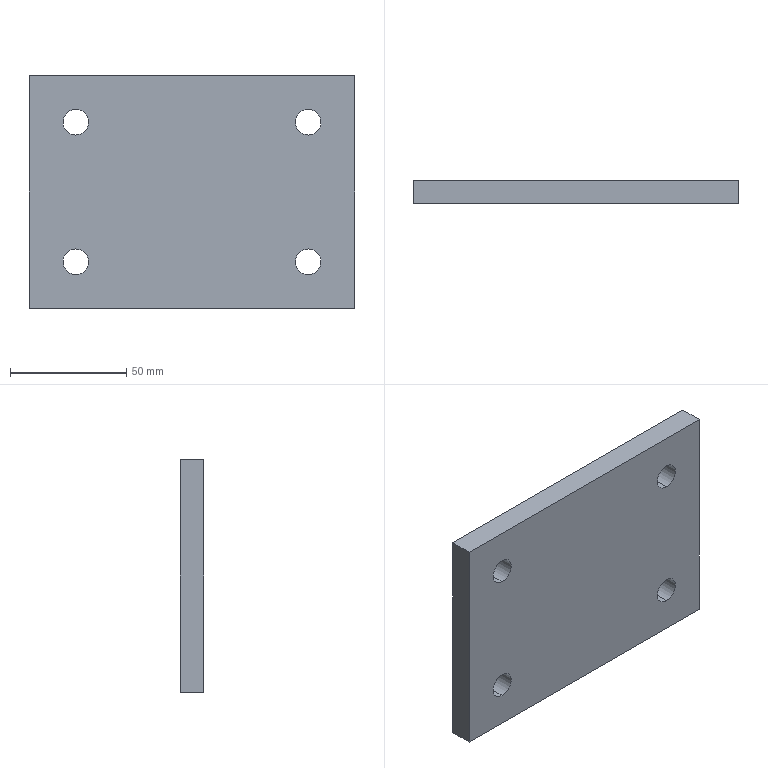Component | SolidWorks | GuardrailMountingPlate-1 | 1 solid | 14 faces | box 140 x 10 x 100 mm | volume 136199 mm3 | cylinder 8 | plane 6 | commonest cylinder face diameters 11 x8 | material Plain Carbon Steel
STEP:
#1=COLOUR_RGB('',0.7922,0.8196,0.9333);
#2=FILL_AREA_STYLE_COLOUR('',#1);
#3=FILL_AREA_STYLE('',(#2));
#4=SURFACE_STYLE_FILL_AREA(#3);
#5=SURFACE_SIDE_STYLE('',(#4));
#6=SURFACE_STYLE_USAGE(.BOTH.,#5);
#7=PRESENTATION_STYLE_ASSIGNMENT((#6));
#8=CARTESIAN_POINT('',(-131.976,-23.964,222.853));
#9=VERTEX_POINT('',#8);
#10=CARTESIAN_POINT('',(-131.976,-23.964,223.286));
#11=VERTEX_POINT('',#10);
#12=CARTESIAN_POINT('',(-131.976,-23.964,223.07));
#13=DIRECTION('',(0.,1.,0.));
#14=DIRECTION('',(0.,0.,1.));
#15=AXIS2_PLACEMENT_3D('',#12,#13,#14);
#16=CIRCLE('',#15,0.2165);
#17=EDGE_CURVE('',#9,#11,#16,.T.);
#18=ORIENTED_EDGE('',*,*,#17,.F.);
#19=CARTESIAN_POINT('',(-131.976,-23.57,222.853));
#20=VERTEX_POINT('',#19);
#21=CARTESIAN_POINT('',(-131.976,-23.964,222.853));
#22=DIRECTION('',(0.,1.,0.));
#23=VECTOR('',#22,39.37);
#24=LINE('',#21,#23);
#25=EDGE_CURVE('',#9,#20,#24,.T.);
#26=ORIENTED_EDGE('',*,*,#25,.T.);
#27=CARTESIAN_POINT('',(-131.976,-23.57,223.286));
#28=VERTEX_POINT('',#27);
#29=CARTESIAN_POINT('',(-131.976,-23.57,223.07));
#30=DIRECTION('',(0.,1.,0.));
#31=DIRECTION('',(0.,0.,1.));
#32=AXIS2_PLACEMENT_3D('',#29,#30,#31);
#33=CIRCLE('',#32,0.2165);
#34=EDGE_CURVE('',#20,#28,#33,.T.);
#35=ORIENTED_EDGE('',*,*,#34,.T.);
#36=CARTESIAN_POINT('',(-131.976,-23.964,223.286));
#37=DIRECTION('',(0.,1.,0.));
#38=VECTOR('',#37,39.37);
#39=LINE('',#36,#38);
#40=EDGE_CURVE('',#11,#28,#39,.T.);
#41=ORIENTED_EDGE('',*,*,#40,.F.);
#42=EDGE_LOOP('',(#18,#26,#35,#41));
#43=FACE_OUTER_BOUND('',#42,.T.);
#44=CARTESIAN_POINT('',(-131.976,-23.964,223.07));
#45=DIRECTION('',(0.,1.,0.));
#46=DIRECTION('',(0.,0.,1.));
#47=AXIS2_PLACEMENT_3D('',#44,#45,#46);
#48=CYLINDRICAL_SURFACE('',#47,0.2165);
#49=ADVANCED_FACE('',(#43),#48,.F.);
#50=CARTESIAN_POINT('',(-128.039,-23.964,222.853));
#51=VERTEX_POINT('',#50);
#52=CARTESIAN_POINT('',(-128.039,-23.964,223.286));
#53=VERTEX_POINT('',#52);
#54=CARTESIAN_POINT('',(-128.039,-23.964,223.07));
#55=DIRECTION('',(0.,1.,0.));
#56=DIRECTION('',(0.,0.,1.));
#57=AXIS2_PLACEMENT_3D('',#54,#55,#56);
#58=CIRCLE('',#57,0.2165);
#59=EDGE_CURVE('',#51,#53,#58,.T.);
#60=ORIENTED_EDGE('',*,*,#59,.F.);
#61=CARTESIAN_POINT('',(-128.039,-23.57,222.853));
#62=VERTEX_POINT('',#61);
#63=CARTESIAN_POINT('',(-128.039,-23.964,222.853));
#64=DIRECTION('',(0.,1.,0.));
#65=VECTOR('',#64,39.37);
#66=LINE('',#63,#65);
#67=EDGE_CURVE('',#51,#62,#66,.T.);
#68=ORIENTED_EDGE('',*,*,#67,.T.);
#69=CARTESIAN_POINT('',(-128.039,-23.57,223.286));
#70=VERTEX_POINT('',#69);
#71=CARTESIAN_POINT('',(-128.039,-23.57,223.07));
#72=DIRECTION('',(0.,1.,0.));
#73=DIRECTION('',(0.,0.,1.));
#74=AXIS2_PLACEMENT_3D('',#71,#72,#73);
#75=CIRCLE('',#74,0.2165);
#76=EDGE_CURVE('',#62,#70,#75,.T.);
#77=ORIENTED_EDGE('',*,*,#76,.T.);
#78=CARTESIAN_POINT('',(-128.039,-23.964,223.286));
#79=DIRECTION('',(0.,1.,0.));
#80=VECTOR('',#79,39.37);
#81=LINE('',#78,#80);
#82=EDGE_CURVE('',#53,#70,#81,.T.);
#83=ORIENTED_EDGE('',*,*,#82,.F.);
#84=EDGE_LOOP('',(#60,#68,#77,#83));
#85=FACE_OUTER_BOUND('',#84,.T.);
#86=CARTESIAN_POINT('',(-128.039,-23.964,223.07));
#87=DIRECTION('',(0.,1.,0.));
#88=DIRECTION('',(0.,0.,1.));
#89=AXIS2_PLACEMENT_3D('',#86,#87,#88);
#90=CYLINDRICAL_SURFACE('',#89,0.2165);
#91=ADVANCED_FACE('',(#85),#90,.F.);
#92=CARTESIAN_POINT('',(-128.039,-23.964,220.491));
#93=VERTEX_POINT('',#92);
#94=CARTESIAN_POINT('',(-128.039,-23.964,220.924));
#95=VERTEX_POINT('',#94);
#96=CARTESIAN_POINT('',(-128.039,-23.964,220.708));
#97=DIRECTION('',(0.,1.,0.));
#98=DIRECTION('',(0.,0.,1.));
#99=AXIS2_PLACEMENT_3D('',#96,#97,#98);
#100=CIRCLE('',#99,0.2165);
#101=EDGE_CURVE('',#93,#95,#100,.T.);
#102=ORIENTED_EDGE('',*,*,#101,.F.);
#103=CARTESIAN_POINT('',(-128.039,-23.57,220.491));
#104=VERTEX_POINT('',#103);
#105=CARTESIAN_POINT('',(-128.039,-23.964,220.491));
#106=DIRECTION('',(0.,1.,0.));
#107=VECTOR('',#106,39.37);
#108=LINE('',#105,#107);
#109=EDGE_CURVE('',#93,#104,#108,.T.);
#110=ORIENTED_EDGE('',*,*,#109,.T.);
#111=CARTESIAN_POINT('',(-128.039,-23.57,220.924));
#112=VERTEX_POINT('',#111);
#113=CARTESIAN_POINT('',(-128.039,-23.57,220.708));
#114=DIRECTION('',(0.,1.,0.));
#115=DIRECTION('',(0.,0.,1.));
#116=AXIS2_PLACEMENT_3D('',#113,#114,#115);
#117=CIRCLE('',#116,0.2165);
#118=EDGE_CURVE('',#104,#112,#117,.T.);
#119=ORIENTED_EDGE('',*,*,#118,.T.);
#120=CARTESIAN_POINT('',(-128.039,-23.964,220.924));
#121=DIRECTION('',(0.,1.,0.));
#122=VECTOR('',#121,39.37);
#123=LINE('',#120,#122);
#124=EDGE_CURVE('',#95,#112,#123,.T.);
#125=ORIENTED_EDGE('',*,*,#124,.F.);
#126=EDGE_LOOP('',(#102,#110,#119,#125));
#127=FACE_OUTER_BOUND('',#126,.T.);
#128=CARTESIAN_POINT('',(-128.039,-23.964,220.708));
#129=DIRECTION('',(0.,1.,0.));
#130=DIRECTION('',(0.,0.,1.));
#131=AXIS2_PLACEMENT_3D('',#128,#129,#130);
#132=CYLINDRICAL_SURFACE('',#131,0.2165);
#133=ADVANCED_FACE('',(#127),#132,.F.);
#134=CARTESIAN_POINT('',(-131.976,-23.964,220.491));
#135=VERTEX_POINT('',#134);
#136=CARTESIAN_POINT('',(-131.976,-23.964,220.924));
#137=VERTEX_POINT('',#136);
#138=CARTESIAN_POINT('',(-131.976,-23.964,220.708));
#139=DIRECTION('',(0.,1.,0.));
#140=DIRECTION('',(0.,0.,1.));
#141=AXIS2_PLACEMENT_3D('',#138,#139,#140);
#142=CIRCLE('',#141,0.2165);
#143=EDGE_CURVE('',#135,#137,#142,.T.);
#144=ORIENTED_EDGE('',*,*,#143,.F.);
#145=CARTESIAN_POINT('',(-131.976,-23.57,220.491));
#146=VERTEX_POINT('',#145);
#147=CARTESIAN_POINT('',(-131.976,-23.964,220.491));
#148=DIRECTION('',(0.,1.,0.));
#149=VECTOR('',#148,39.37);
#150=LINE('',#147,#149);
#151=EDGE_CURVE('',#135,#146,#150,.T.);
#152=ORIENTED_EDGE('',*,*,#151,.T.);
#153=CARTESIAN_POINT('',(-131.976,-23.57,220.924));
#154=VERTEX_POINT('',#153);
#155=CARTESIAN_POINT('',(-131.976,-23.57,220.708));
#156=DIRECTION('',(0.,1.,0.));
#157=DIRECTION('',(0.,0.,1.));
#158=AXIS2_PLACEMENT_3D('',#155,#156,#157);
#159=CIRCLE('',#158,0.2165);
#160=EDGE_CURVE('',#146,#154,#159,.T.);
#161=ORIENTED_EDGE('',*,*,#160,.T.);
#162=CARTESIAN_POINT('',(-131.976,-23.964,220.924));
#163=DIRECTION('',(0.,1.,0.));
#164=VECTOR('',#163,39.37);
#165=LINE('',#162,#164);
#166=EDGE_CURVE('',#137,#154,#165,.T.);
#167=ORIENTED_EDGE('',*,*,#166,.F.);
#168=EDGE_LOOP('',(#144,#152,#161,#167));
#169=FACE_OUTER_BOUND('',#168,.T.);
#170=CARTESIAN_POINT('',(-131.976,-23.964,220.708));
#171=DIRECTION('',(0.,1.,0.));
#172=DIRECTION('',(0.,0.,1.));
#173=AXIS2_PLACEMENT_3D('',#170,#171,#172);
#174=CYLINDRICAL_SURFACE('',#173,0.2165);
#175=ADVANCED_FACE('',(#169),#174,.F.);
#176=CARTESIAN_POINT('',(-127.252,-23.57,223.857));
#177=VERTEX_POINT('',#176);
#178=CARTESIAN_POINT('',(-127.252,-23.57,219.92));
#179=VERTEX_POINT('',#178);
#180=CARTESIAN_POINT('',(-127.252,-23.57,219.92));
#181=DIRECTION('',(0.,0.,-1.));
#182=VECTOR('',#181,39.37);
#183=LINE('',#180,#182);
#184=EDGE_CURVE('',#177,#179,#183,.T.);
#185=ORIENTED_EDGE('',*,*,#184,.F.);
#186=CARTESIAN_POINT('',(-127.252,-23.964,223.857));
#187=VERTEX_POINT('',#186);
#188=CARTESIAN_POINT('',(-127.252,-23.964,223.857));
#189=DIRECTION('',(0.,1.,0.));
#190=VECTOR('',#189,39.37);
#191=LINE('',#188,#190);
#192=EDGE_CURVE('',#187,#177,#191,.T.);
#193=ORIENTED_EDGE('',*,*,#192,.F.);
#194=CARTESIAN_POINT('',(-127.252,-23.964,219.92));
#195=VERTEX_POINT('',#194);
#196=CARTESIAN_POINT('',(-127.252,-23.964,219.92));
#197=DIRECTION('',(0.,0.,-1.));
#198=VECTOR('',#197,39.37);
#199=LINE('',#196,#198);
#200=EDGE_CURVE('',#187,#195,#199,.T.);
#201=ORIENTED_EDGE('',*,*,#200,.T.);
#202=CARTESIAN_POINT('',(-127.252,-23.964,219.92));
#203=DIRECTION('',(0.,1.,0.));
#204=VECTOR('',#203,39.37);
#205=LINE('',#202,#204);
#206=EDGE_CURVE('',#195,#179,#205,.T.);
#207=ORIENTED_EDGE('',*,*,#206,.T.);
#208=EDGE_LOOP('',(#185,#193,#201,#207));
#209=FACE_OUTER_BOUND('',#208,.T.);
#210=CARTESIAN_POINT('',(-127.252,-23.964,219.92));
#211=DIRECTION('',(1.,0.,0.));
#212=DIRECTION('',(0.,0.,-1.));
#213=AXIS2_PLACEMENT_3D('',#210,#211,#212);
#214=PLANE('',#213);
#215=ADVANCED_FACE('',(#209),#214,.T.);
#216=CARTESIAN_POINT('',(-132.764,-23.57,223.857));
#217=VERTEX_POINT('',#216);
#218=CARTESIAN_POINT('',(-132.764,-23.57,223.857));
#219=DIRECTION('',(1.,0.,0.));
#220=VECTOR('',#219,39.37);
#221=LINE('',#218,#220);
#222=EDGE_CURVE('',#217,#177,#221,.T.);
#223=ORIENTED_EDGE('',*,*,#222,.F.);
#224=CARTESIAN_POINT('',(-132.764,-23.964,223.857));
#225=VERTEX_POINT('',#224);
#226=CARTESIAN_POINT('',(-132.764,-23.964,223.857));
#227=DIRECTION('',(0.,1.,0.));
#228=VECTOR('',#227,39.37);
#229=LINE('',#226,#228);
#230=EDGE_CURVE('',#225,#217,#229,.T.);
#231=ORIENTED_EDGE('',*,*,#230,.F.);
#232=CARTESIAN_POINT('',(-132.764,-23.964,223.857));
#233=DIRECTION('',(1.,0.,0.));
#234=VECTOR('',#233,39.37);
#235=LINE('',#232,#234);
#236=EDGE_CURVE('',#225,#187,#235,.T.);
#237=ORIENTED_EDGE('',*,*,#236,.T.);
#238=ORIENTED_EDGE('',*,*,#192,.T.);
#239=EDGE_LOOP('',(#223,#231,#237,#238));
#240=FACE_OUTER_BOUND('',#239,.T.);
#241=CARTESIAN_POINT('',(-132.764,-23.964,223.857));
#242=DIRECTION('',(0.,0.,1.));
#243=DIRECTION('',(1.,0.,0.));
#244=AXIS2_PLACEMENT_3D('',#241,#242,#243);
#245=PLANE('',#244);
#246=ADVANCED_FACE('',(#240),#245,.T.);
#247=CARTESIAN_POINT('',(-132.764,-23.57,219.92));
#248=VERTEX_POINT('',#247);
#249=CARTESIAN_POINT('',(-132.764,-23.57,219.92));
#250=DIRECTION('',(0.,0.,1.));
#251=VECTOR('',#250,39.37);
#252=LINE('',#249,#251);
#253=EDGE_CURVE('',#248,#217,#252,.T.);
#254=ORIENTED_EDGE('',*,*,#253,.F.);
#255=CARTESIAN_POINT('',(-132.764,-23.964,219.92));
#256=VERTEX_POINT('',#255);
#257=CARTESIAN_POINT('',(-132.764,-23.964,219.92));
#258=DIRECTION('',(0.,1.,0.));
#259=VECTOR('',#258,39.37);
#260=LINE('',#257,#259);
#261=EDGE_CURVE('',#256,#248,#260,.T.);
#262=ORIENTED_EDGE('',*,*,#261,.F.);
#263=CARTESIAN_POINT('',(-132.764,-23.964,219.92));
#264=DIRECTION('',(0.,0.,1.));
#265=VECTOR('',#264,39.37);
#266=LINE('',#263,#265);
#267=EDGE_CURVE('',#256,#225,#266,.T.);
#268=ORIENTED_EDGE('',*,*,#267,.T.);
#269=ORIENTED_EDGE('',*,*,#230,.T.);
#270=EDGE_LOOP('',(#254,#262,#268,#269));
#271=FACE_OUTER_BOUND('',#270,.T.);
#272=CARTESIAN_POINT('',(-132.764,-23.964,219.92));
#273=DIRECTION('',(-1.,0.,0.));
#274=DIRECTION('',(0.,0.,1.));
#275=AXIS2_PLACEMENT_3D('',#272,#273,#274);
#276=PLANE('',#275);
#277=ADVANCED_FACE('',(#271),#276,.T.);
#278=CARTESIAN_POINT('',(-132.764,-23.57,219.92));
#279=DIRECTION('',(-1.,0.,0.));
#280=VECTOR('',#279,39.37);
#281=LINE('',#278,#280);
#282=EDGE_CURVE('',#179,#248,#281,.T.);
#283=ORIENTED_EDGE('',*,*,#282,.F.);
#284=ORIENTED_EDGE('',*,*,#206,.F.);
#285=CARTESIAN_POINT('',(-132.764,-23.964,219.92));
#286=DIRECTION('',(-1.,0.,0.));
#287=VECTOR('',#286,39.37);
#288=LINE('',#285,#287);
#289=EDGE_CURVE('',#195,#256,#288,.T.);
#290=ORIENTED_EDGE('',*,*,#289,.T.);
#291=ORIENTED_EDGE('',*,*,#261,.T.);
#292=EDGE_LOOP('',(#283,#284,#290,#291));
#293=FACE_OUTER_BOUND('',#292,.T.);
#294=CARTESIAN_POINT('',(-132.764,-23.964,219.92));
#295=DIRECTION('',(0.,0.,-1.));
#296=DIRECTION('',(-1.,0.,0.));
#297=AXIS2_PLACEMENT_3D('',#294,#295,#296);
#298=PLANE('',#297);
#299=ADVANCED_FACE('',(#293),#298,.T.);
#300=CARTESIAN_POINT('',(-131.976,-23.964,223.07));
#301=DIRECTION('',(0.,1.,0.));
#302=DIRECTION('',(0.,0.,1.));
#303=AXIS2_PLACEMENT_3D('',#300,#301,#302);
#304=CIRCLE('',#303,0.2165);
#305=EDGE_CURVE('',#11,#9,#304,.T.);
#306=ORIENTED_EDGE('',*,*,#305,.T.);
#307=ORIENTED_EDGE('',*,*,#17,.T.);
#308=EDGE_LOOP('',(#306,#307));
#309=FACE_BOUND('',#308,.T.);
#310=CARTESIAN_POINT('',(-128.039,-23.964,223.07));
#311=DIRECTION('',(0.,1.,0.));
#312=DIRECTION('',(0.,0.,1.));
#313=AXIS2_PLACEMENT_3D('',#310,#311,#312);
#314=CIRCLE('',#313,0.2165);
#315=EDGE_CURVE('',#53,#51,#314,.T.);
#316=ORIENTED_EDGE('',*,*,#315,.T.);
#317=ORIENTED_EDGE('',*,*,#59,.T.);
#318=EDGE_LOOP('',(#316,#317));
#319=FACE_BOUND('',#318,.T.);
#320=CARTESIAN_POINT('',(-128.039,-23.964,220.708));
#321=DIRECTION('',(0.,1.,0.));
#322=DIRECTION('',(0.,0.,1.));
#323=AXIS2_PLACEMENT_3D('',#320,#321,#322);
#324=CIRCLE('',#323,0.2165);
#325=EDGE_CURVE('',#95,#93,#324,.T.);
#326=ORIENTED_EDGE('',*,*,#325,.T.);
#327=ORIENTED_EDGE('',*,*,#101,.T.);
#328=EDGE_LOOP('',(#326,#327));
#329=FACE_BOUND('',#328,.T.);
#330=CARTESIAN_POINT('',(-131.976,-23.964,220.708));
#331=DIRECTION('',(0.,1.,0.));
#332=DIRECTION('',(0.,0.,1.));
#333=AXIS2_PLACEMENT_3D('',#330,#331,#332);
#334=CIRCLE('',#333,0.2165);
#335=EDGE_CURVE('',#137,#135,#334,.T.);
#336=ORIENTED_EDGE('',*,*,#335,.T.);
#337=ORIENTED_EDGE('',*,*,#143,.T.);
#338=EDGE_LOOP('',(#336,#337));
#339=FACE_BOUND('',#338,.T.);
#340=ORIENTED_EDGE('',*,*,#200,.F.);
#341=ORIENTED_EDGE('',*,*,#236,.F.);
#342=ORIENTED_EDGE('',*,*,#267,.F.);
#343=ORIENTED_EDGE('',*,*,#289,.F.);
#344=EDGE_LOOP('',(#340,#341,#342,#343));
#345=FACE_OUTER_BOUND('',#344,.T.);
#346=CARTESIAN_POINT('',(-132.764,-23.964,219.92));
#347=DIRECTION('',(0.,1.,0.));
#348=DIRECTION('',(0.,0.,1.));
#349=AXIS2_PLACEMENT_3D('',#346,#347,#348);
#350=PLANE('',#349);
#351=ADVANCED_FACE('',(#309,#319,#329,#339,#345),#350,.F.);
#352=CARTESIAN_POINT('',(-131.976,-23.57,223.07));
#353=DIRECTION('',(0.,1.,0.));
#354=DIRECTION('',(0.,0.,1.));
#355=AXIS2_PLACEMENT_3D('',#352,#353,#354);
#356=CIRCLE('',#355,0.2165);
#357=EDGE_CURVE('',#28,#20,#356,.T.);
#358=ORIENTED_EDGE('',*,*,#357,.F.);
#359=ORIENTED_EDGE('',*,*,#34,.F.);
#360=EDGE_LOOP('',(#358,#359));
#361=FACE_BOUND('',#360,.T.);
#362=CARTESIAN_POINT('',(-128.039,-23.57,223.07));
#363=DIRECTION('',(0.,1.,0.));
#364=DIRECTION('',(0.,0.,1.));
#365=AXIS2_PLACEMENT_3D('',#362,#363,#364);
#366=CIRCLE('',#365,0.2165);
#367=EDGE_CURVE('',#70,#62,#366,.T.);
#368=ORIENTED_EDGE('',*,*,#367,.F.);
#369=ORIENTED_EDGE('',*,*,#76,.F.);
#370=EDGE_LOOP('',(#368,#369));
#371=FACE_BOUND('',#370,.T.);
#372=CARTESIAN_POINT('',(-128.039,-23.57,220.708));
#373=DIRECTION('',(0.,1.,0.));
#374=DIRECTION('',(0.,0.,1.));
#375=AXIS2_PLACEMENT_3D('',#372,#373,#374);
#376=CIRCLE('',#375,0.2165);
#377=EDGE_CURVE('',#112,#104,#376,.T.);
#378=ORIENTED_EDGE('',*,*,#377,.F.);
#379=ORIENTED_EDGE('',*,*,#118,.F.);
#380=EDGE_LOOP('',(#378,#379));
#381=FACE_BOUND('',#380,.T.);
#382=CARTESIAN_POINT('',(-131.976,-23.57,220.708));
#383=DIRECTION('',(0.,1.,0.));
#384=DIRECTION('',(0.,0.,1.));
#385=AXIS2_PLACEMENT_3D('',#382,#383,#384);
#386=CIRCLE('',#385,0.2165);
#387=EDGE_CURVE('',#154,#146,#386,.T.);
#388=ORIENTED_EDGE('',*,*,#387,.F.);
#389=ORIENTED_EDGE('',*,*,#160,.F.);
#390=EDGE_LOOP('',(#388,#389));
#391=FACE_BOUND('',#390,.T.);
#392=ORIENTED_EDGE('',*,*,#184,.T.);
#393=ORIENTED_EDGE('',*,*,#282,.T.);
#394=ORIENTED_EDGE('',*,*,#253,.T.);
#395=ORIENTED_EDGE('',*,*,#222,.T.);
#396=EDGE_LOOP('',(#392,#393,#394,#395));
#397=FACE_OUTER_BOUND('',#396,.T.);
#398=CARTESIAN_POINT('',(-132.764,-23.57,219.92));
#399=DIRECTION('',(0.,1.,0.));
#400=DIRECTION('',(0.,0.,1.));
#401=AXIS2_PLACEMENT_3D('',#398,#399,#400);
#402=PLANE('',#401);
#403=ADVANCED_FACE('',(#361,#371,#381,#391,#397),#402,.T.);
#404=ORIENTED_EDGE('',*,*,#151,.F.);
#405=ORIENTED_EDGE('',*,*,#335,.F.);
#406=ORIENTED_EDGE('',*,*,#166,.T.);
#407=ORIENTED_EDGE('',*,*,#387,.T.);
#408=EDGE_LOOP('',(#404,#405,#406,#407));
#409=FACE_OUTER_BOUND('',#408,.T.);
#410=CARTESIAN_POINT('',(-131.976,-23.964,220.708));
#411=DIRECTION('',(0.,1.,0.));
#412=DIRECTION('',(0.,0.,1.));
#413=AXIS2_PLACEMENT_3D('',#410,#411,#412);
#414=CYLINDRICAL_SURFACE('',#413,0.2165);
#415=ADVANCED_FACE('',(#409),#414,.F.);
#416=ORIENTED_EDGE('',*,*,#109,.F.);
#417=ORIENTED_EDGE('',*,*,#325,.F.);
#418=ORIENTED_EDGE('',*,*,#124,.T.);
#419=ORIENTED_EDGE('',*,*,#377,.T.);
#420=EDGE_LOOP('',(#416,#417,#418,#419));
#421=FACE_OUTER_BOUND('',#420,.T.);
#422=CARTESIAN_POINT('',(-128.039,-23.964,220.708));
#423=DIRECTION('',(0.,1.,0.));
#424=DIRECTION('',(0.,0.,1.));
#425=AXIS2_PLACEMENT_3D('',#422,#423,#424);
#426=CYLINDRICAL_SURFACE('',#425,0.2165);
#427=ADVANCED_FACE('',(#421),#426,.F.);
#428=ORIENTED_EDGE('',*,*,#67,.F.);
#429=ORIENTED_EDGE('',*,*,#315,.F.);
#430=ORIENTED_EDGE('',*,*,#82,.T.);
#431=ORIENTED_EDGE('',*,*,#367,.T.);
#432=EDGE_LOOP('',(#428,#429,#430,#431));
#433=FACE_OUTER_BOUND('',#432,.T.);
#434=CARTESIAN_POINT('',(-128.039,-23.964,223.07));
#435=DIRECTION('',(0.,1.,0.));
#436=DIRECTION('',(0.,0.,1.));
#437=AXIS2_PLACEMENT_3D('',#434,#435,#436);
#438=CYLINDRICAL_SURFACE('',#437,0.2165);
#439=ADVANCED_FACE('',(#433),#438,.F.);
#440=ORIENTED_EDGE('',*,*,#25,.F.);
#441=ORIENTED_EDGE('',*,*,#305,.F.);
#442=ORIENTED_EDGE('',*,*,#40,.T.);
#443=ORIENTED_EDGE('',*,*,#357,.T.);
#444=EDGE_LOOP('',(#440,#441,#442,#443));
#445=FACE_OUTER_BOUND('',#444,.T.);
#446=CARTESIAN_POINT('',(-131.976,-23.964,223.07));
#447=DIRECTION('',(0.,1.,0.));
#448=DIRECTION('',(0.,0.,1.));
#449=AXIS2_PLACEMENT_3D('',#446,#447,#448);
#450=CYLINDRICAL_SURFACE('',#449,0.2165);
#451=ADVANCED_FACE('',(#445),#450,.F.);
#452=CLOSED_SHELL('',(#49,#91,#133,#175,#215,#246,#277,#299,#351,#403,#415,#427,#439,#451));
#453=MANIFOLD_SOLID_BREP('',#452);
#454=STYLED_ITEM('',(#7),#453);
#455=PRESENTATION_LAYER_ASSIGNMENT('','',(#454));
#456=(LENGTH_UNIT()NAMED_UNIT(*)SI_UNIT($,.METRE.));
#457=LENGTH_MEASURE_WITH_UNIT(LENGTH_MEASURE(0.0254),#456);
#458=DIMENSIONAL_EXPONENTS(1.,0.,0.,0.,0.,0.,0.);
#459=(CONVERSION_BASED_UNIT('',#457)LENGTH_UNIT()NAMED_UNIT(#458));
#460=UNCERTAINTY_MEASURE_WITH_UNIT(LENGTH_MEASURE(0.00001),#459,'','');
#461=(NAMED_UNIT(*)PLANE_ANGLE_UNIT()SI_UNIT($,.RADIAN.));
#462=(NAMED_UNIT(*)SI_UNIT($,.STERADIAN.)SOLID_ANGLE_UNIT());
#463=(GEOMETRIC_REPRESENTATION_CONTEXT(3)GLOBAL_UNCERTAINTY_ASSIGNED_CONTEXT((#460))GLOBAL_UNIT_ASSIGNED_CONTEXT((#459,#461,#462))REPRESENTATION_CONTEXT('',''));
#464=MECHANICAL_DESIGN_GEOMETRIC_PRESENTATION_REPRESENTATION('',(#454),#463);
#465=CARTESIAN_POINT('',(0.,0.,0.));
#466=DIRECTION('',(0.,0.,1.));
#467=DIRECTION('',(1.,0.,0.));
#468=AXIS2_PLACEMENT_3D('',#465,#466,#467);
#469=(LENGTH_UNIT()NAMED_UNIT(*)SI_UNIT($,.METRE.));
#470=LENGTH_MEASURE_WITH_UNIT(LENGTH_MEASURE(0.0254),#469);
#471=DIMENSIONAL_EXPONENTS(1.,0.,0.,0.,0.,0.,0.);
#472=(CONVERSION_BASED_UNIT('',#470)LENGTH_UNIT()NAMED_UNIT(#471));
#473=UNCERTAINTY_MEASURE_WITH_UNIT(LENGTH_MEASURE(0.00001),#472,'','');
#474=(NAMED_UNIT(*)PLANE_ANGLE_UNIT()SI_UNIT($,.RADIAN.));
#475=(NAMED_UNIT(*)SI_UNIT($,.STERADIAN.)SOLID_ANGLE_UNIT());
#476=(GEOMETRIC_REPRESENTATION_CONTEXT(3)GLOBAL_UNCERTAINTY_ASSIGNED_CONTEXT((#473))GLOBAL_UNIT_ASSIGNED_CONTEXT((#472,#474,#475))REPRESENTATION_CONTEXT('',''));
#477=ADVANCED_BREP_SHAPE_REPRESENTATION('',(#453,#468),#476);